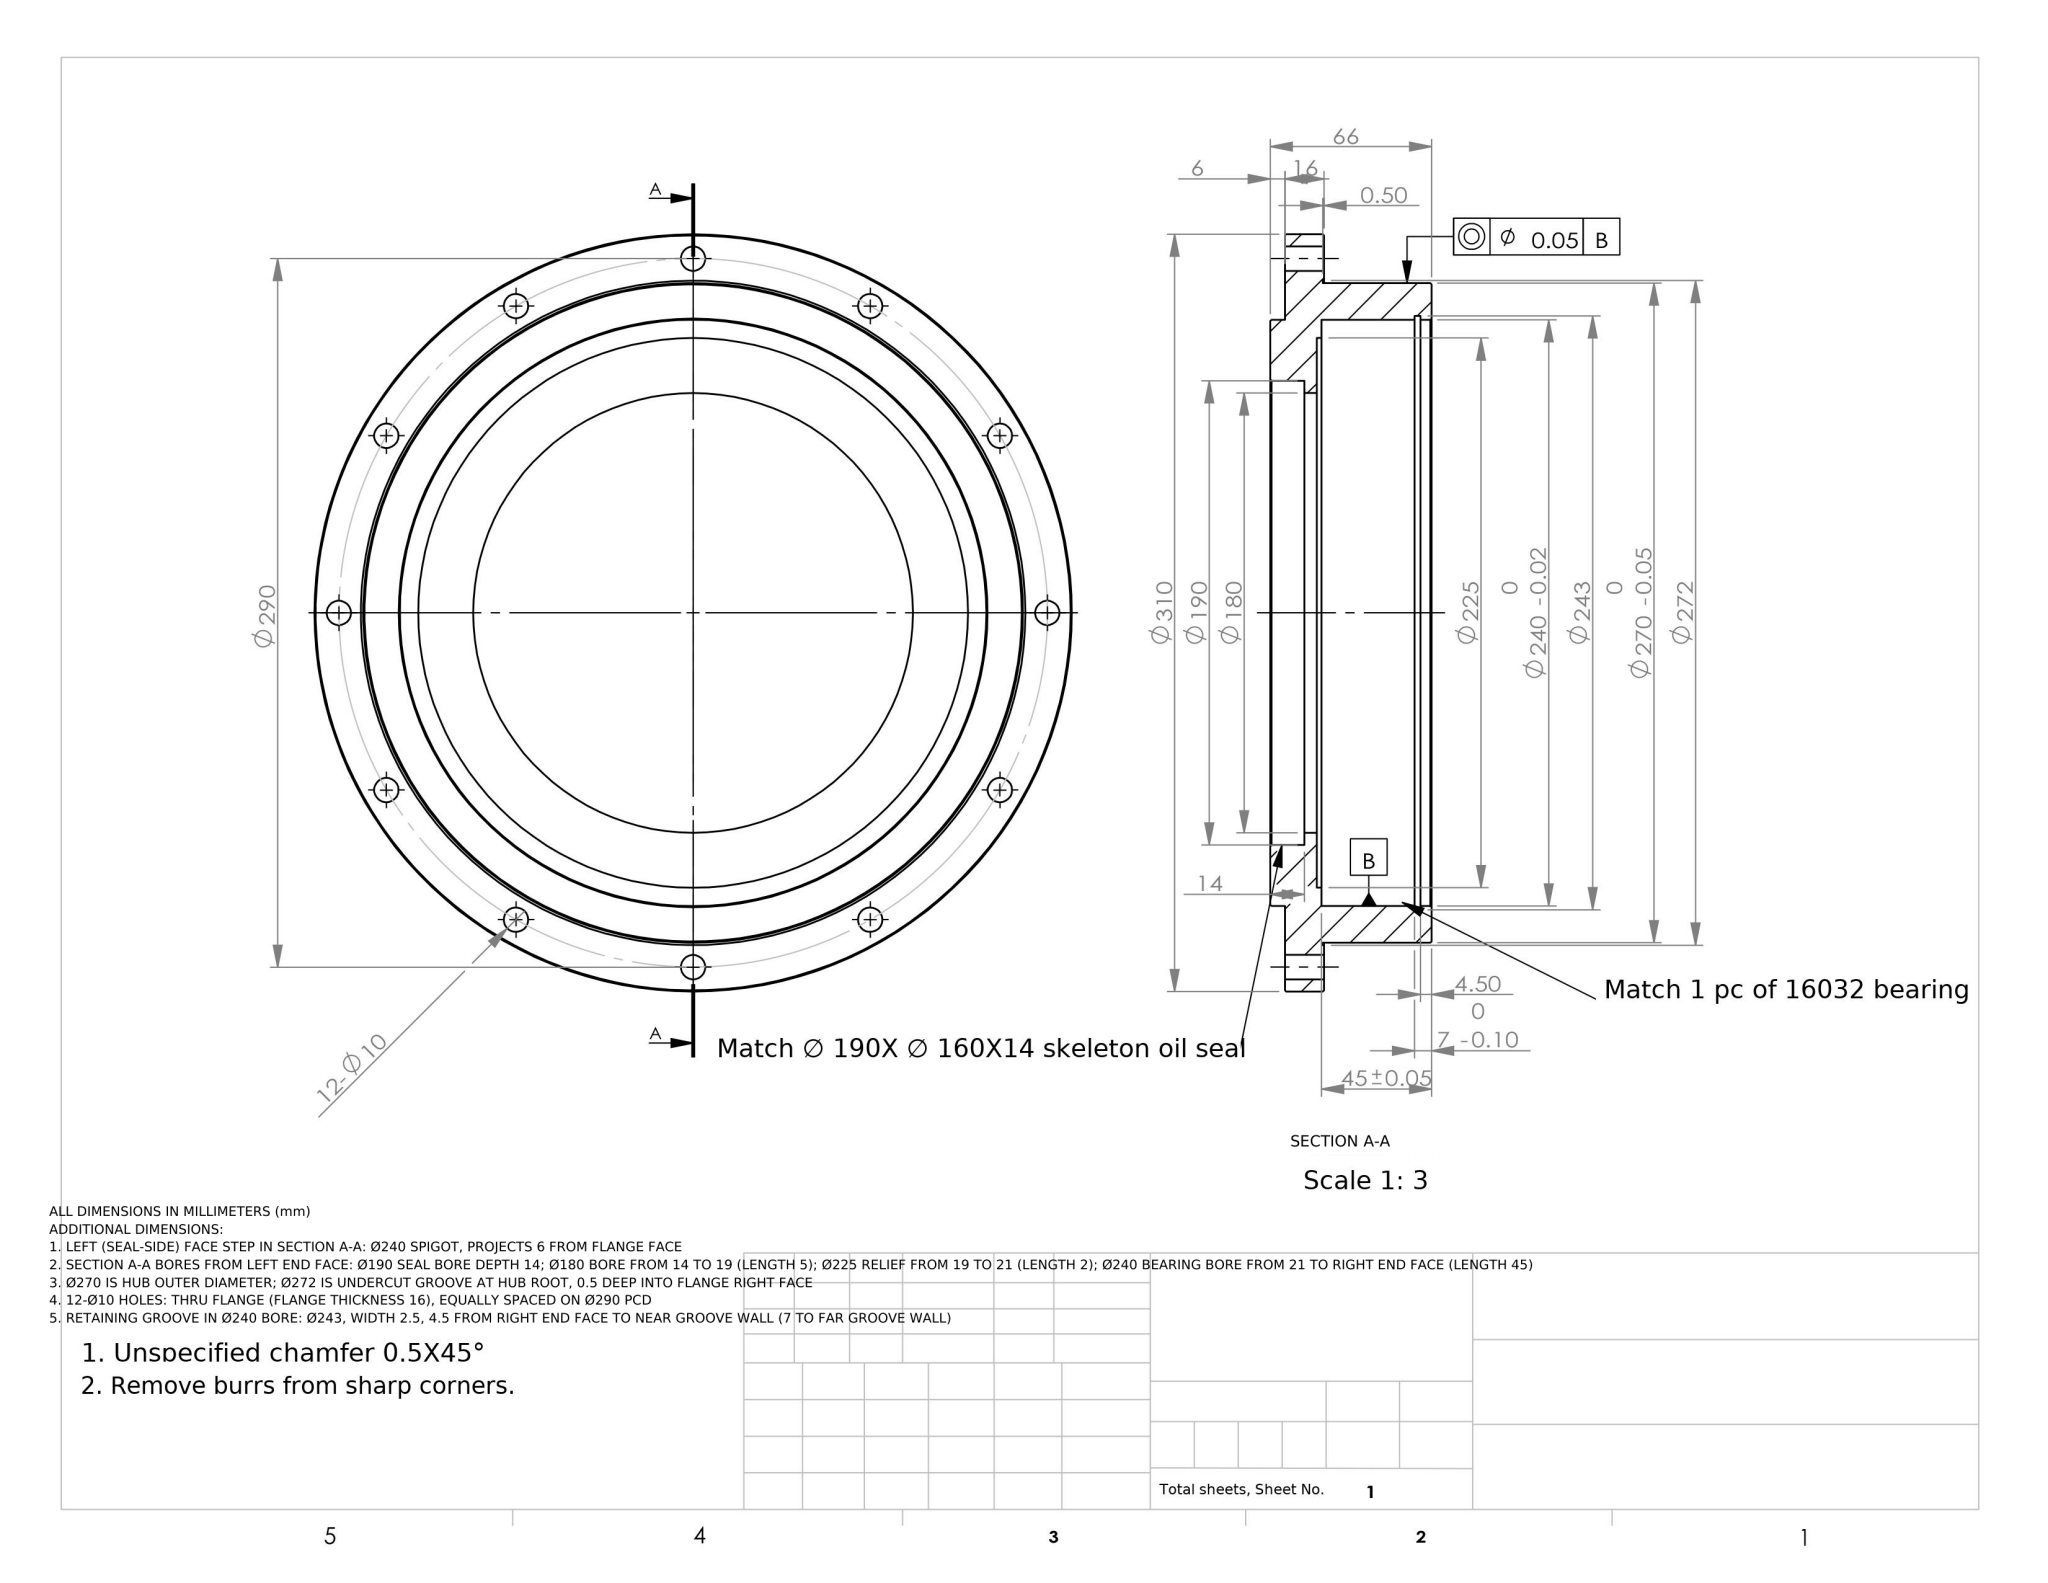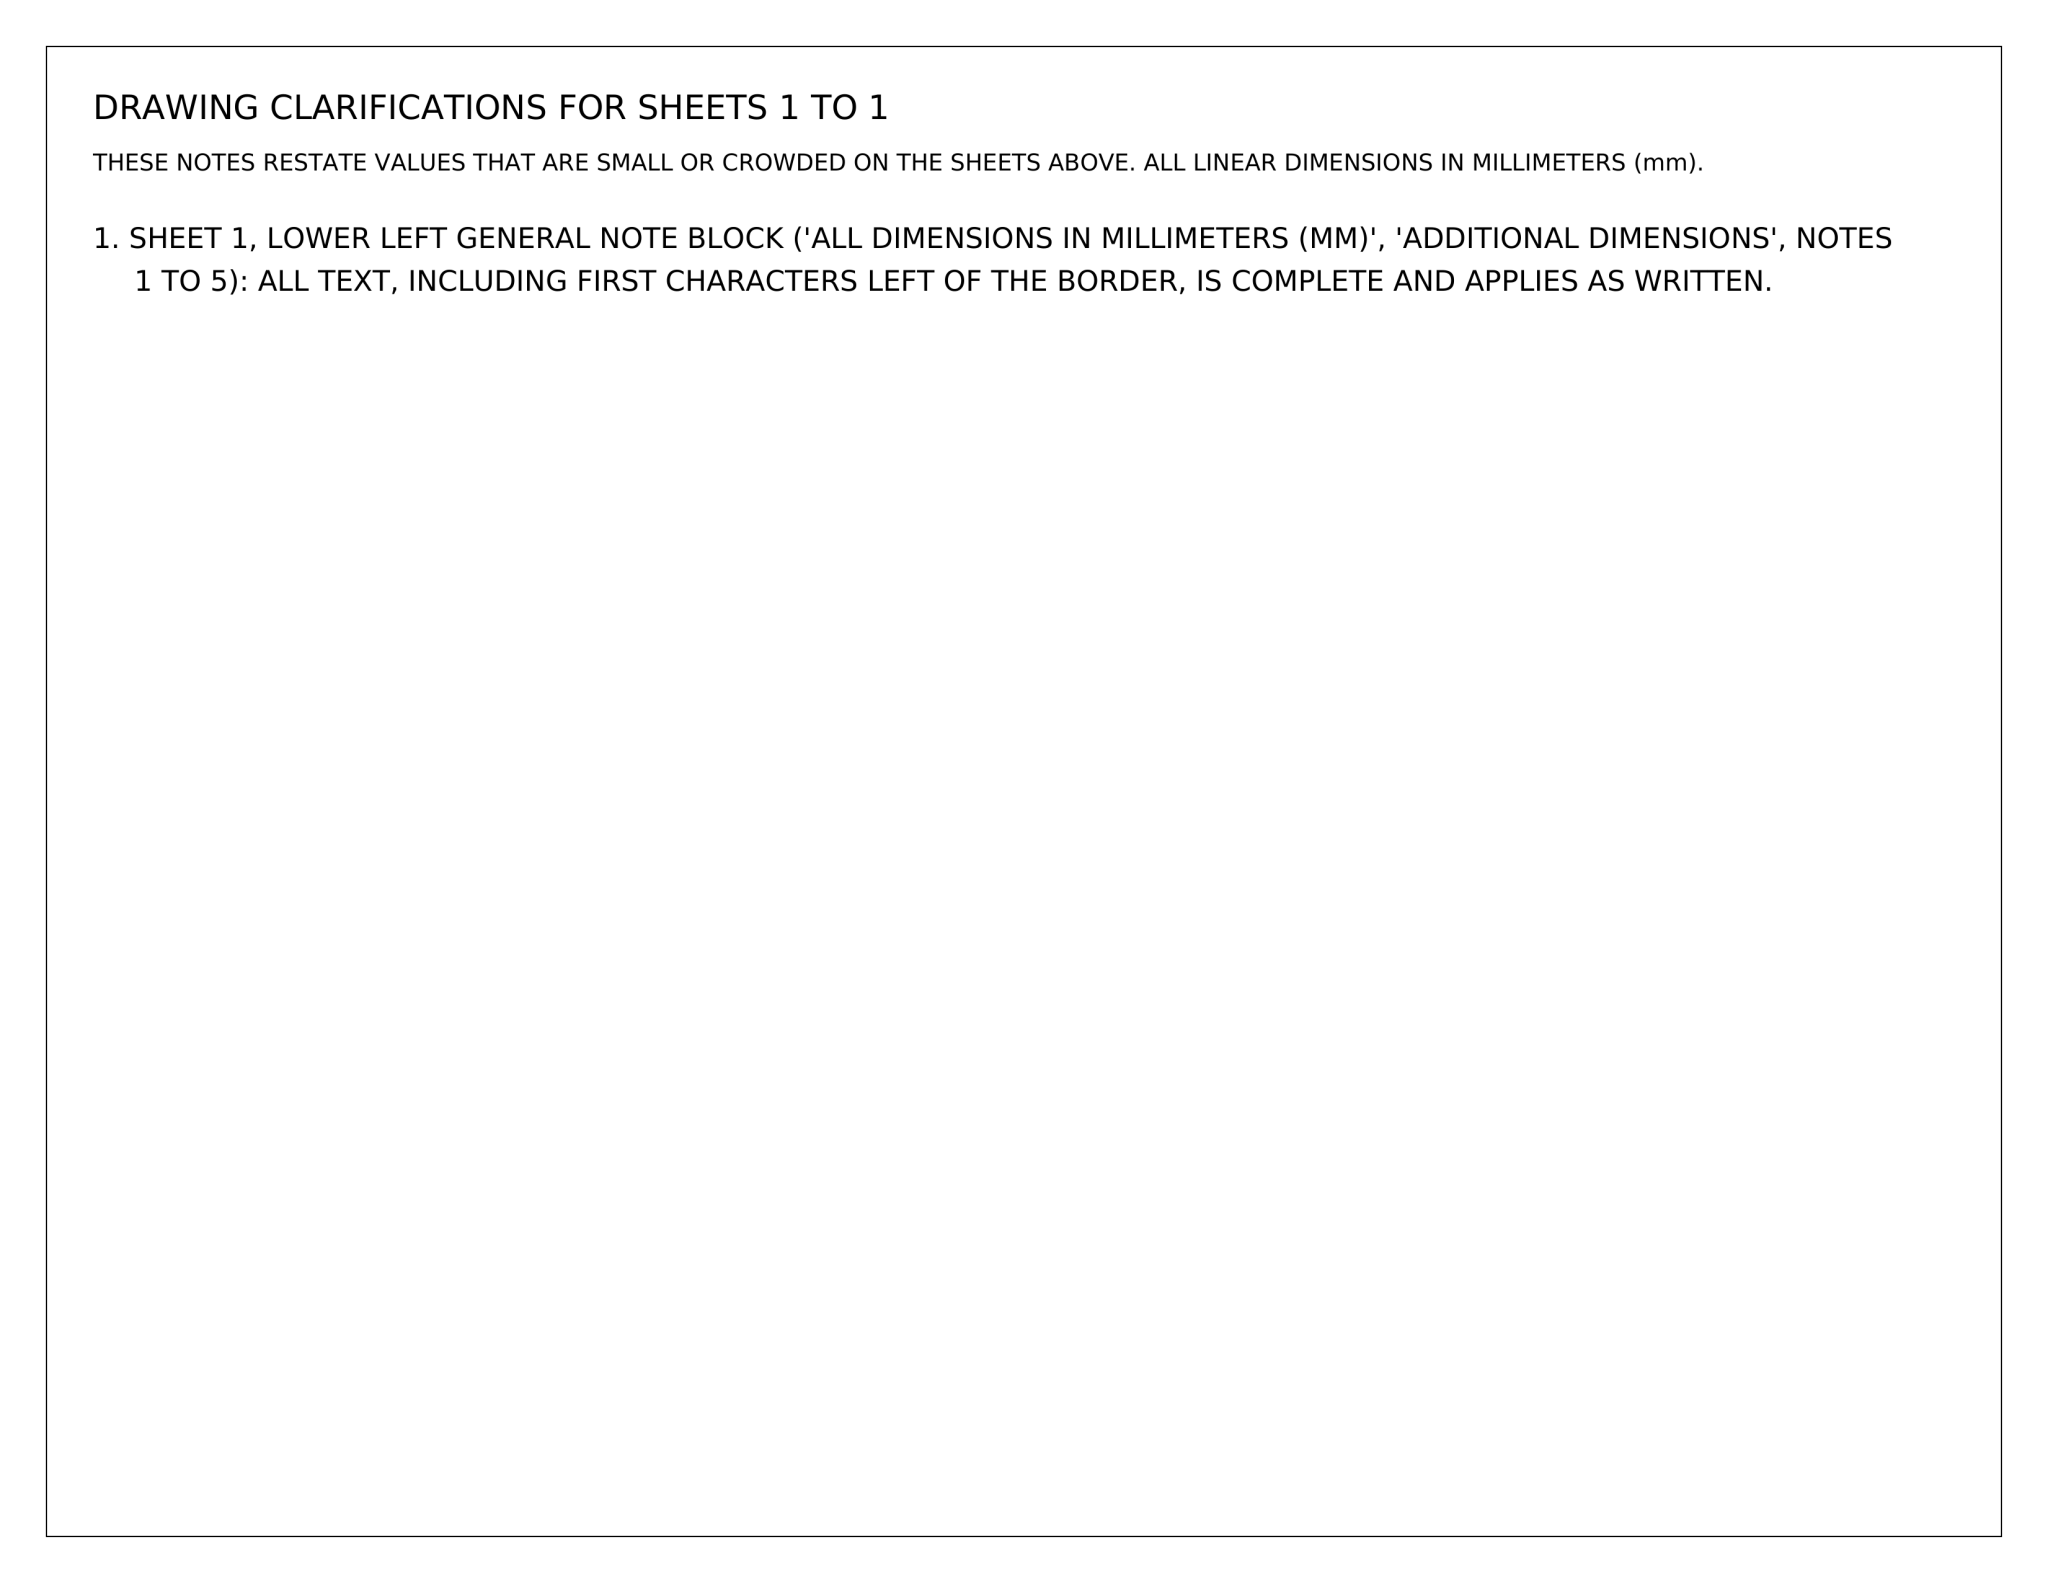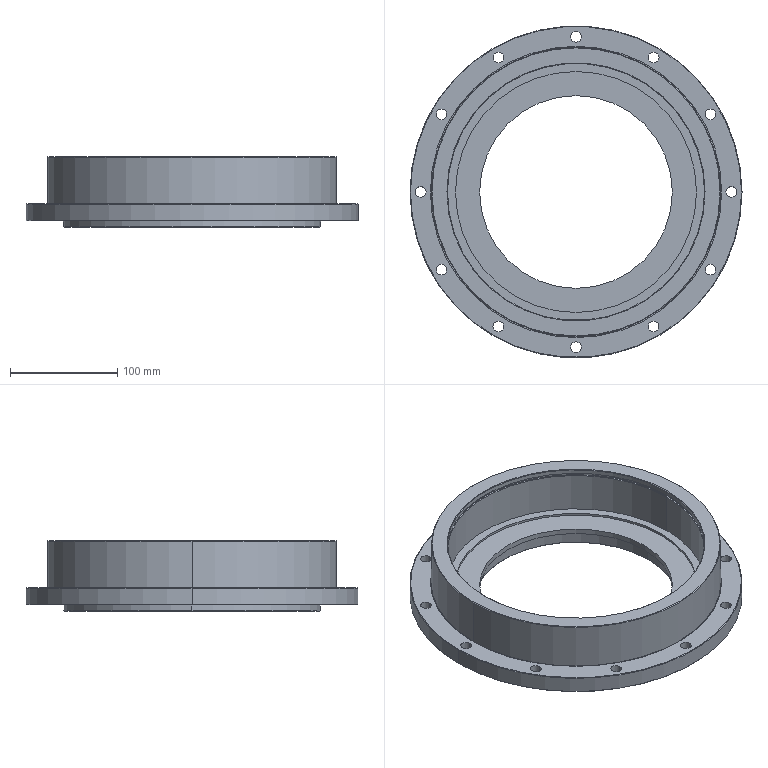Part | NX | mm | 1 solid | 66 faces | box 310 x 310 x 66 mm | volume 1339894 mm3 | cylinder 44 | cone 12 | plane 10 | commonest cylinder face diameters 10 x24 240 x6 272 x2 180 x2 243 x2 270 x2 225 x2 190 x2